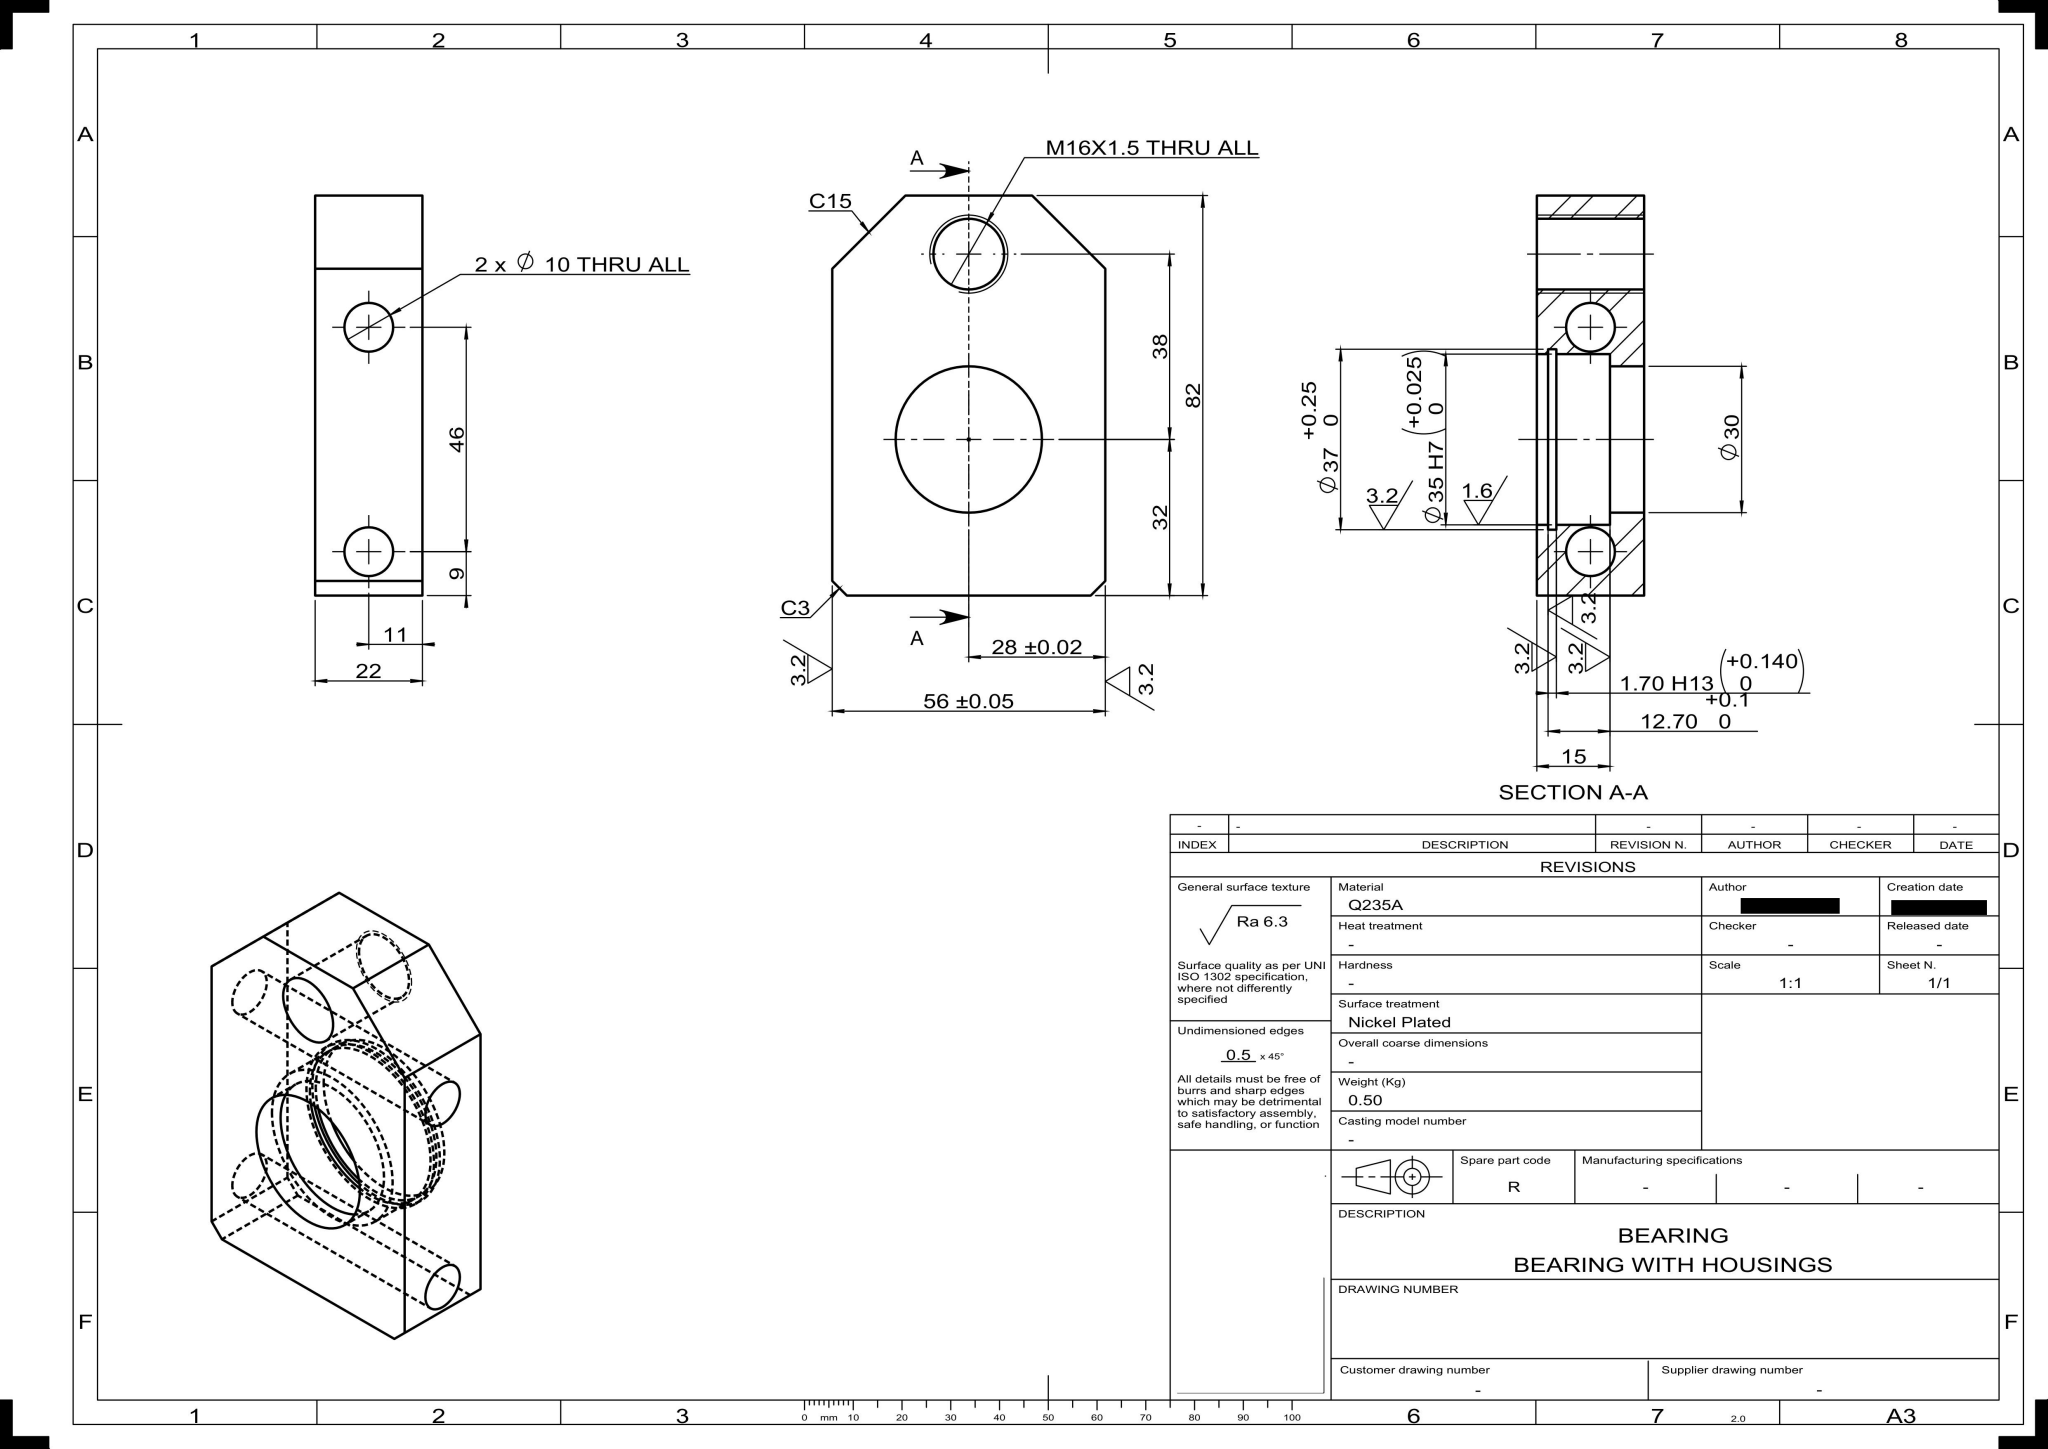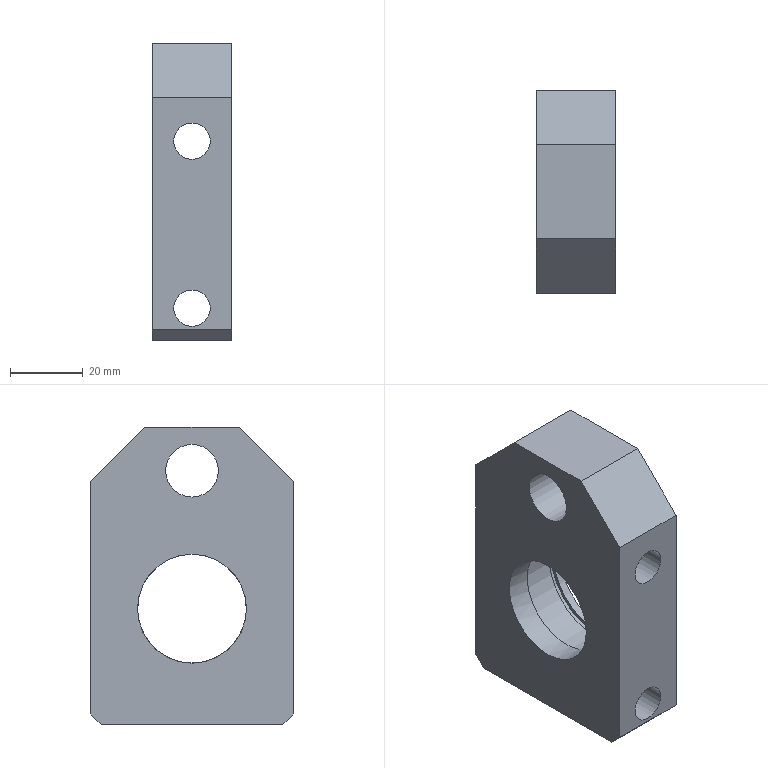Part | NX | mm | 1 solid | 20 faces | box 22 x 56 x 82 mm | volume 63875 mm3 | plane 13 | cylinder 7 | commonest cylinder face diameters 35 x2 10 x2 14.5 x1 30 x1 37 x1
STEP:
#1=CARTESIAN_POINT('',(0.,0.,0.));
#2=DIRECTION('',(0.,0.,1.));
#3=DIRECTION('',(1.,0.,0.));
#4=AXIS2_PLACEMENT_3D('',#1,#2,#3);
#5=(LENGTH_UNIT()NAMED_UNIT(*)SI_UNIT(.MILLI.,.METRE.));
#6=UNCERTAINTY_MEASURE_WITH_UNIT(LENGTH_MEASURE(0.00002),#5,'','');
#7=(NAMED_UNIT(*)PLANE_ANGLE_UNIT()SI_UNIT($,.RADIAN.));
#8=PLANE_ANGLE_MEASURE_WITH_UNIT(PLANE_ANGLE_MEASURE(0.01745),#7);
#9=DIMENSIONAL_EXPONENTS(0.,0.,0.,0.,0.,0.,0.);
#10=(CONVERSION_BASED_UNIT('',#8)NAMED_UNIT(#9)PLANE_ANGLE_UNIT());
#11=(NAMED_UNIT(*)SI_UNIT($,.STERADIAN.)SOLID_ANGLE_UNIT());
#12=(GEOMETRIC_REPRESENTATION_CONTEXT(3)GLOBAL_UNCERTAINTY_ASSIGNED_CONTEXT((#6))GLOBAL_UNIT_ASSIGNED_CONTEXT((#5,#10,#11))REPRESENTATION_CONTEXT('',''));
#13=SHAPE_REPRESENTATION('',(#4),#12);
#14=CARTESIAN_POINT('',(-4.,0.,14.5));
#15=VERTEX_POINT('',#14);
#16=CARTESIAN_POINT('',(-4.,0.,32.));
#17=DIRECTION('',(1.,0.,0.));
#18=DIRECTION('',(0.,0.,-1.));
#19=AXIS2_PLACEMENT_3D('',#16,#17,#18);
#20=CIRCLE('',#19,17.5);
#21=EDGE_CURVE('',#15,#15,#20,.T.);
#22=ORIENTED_EDGE('',*,*,#21,.F.);
#23=EDGE_LOOP('',(#22));
#24=FACE_BOUND('',#23,.T.);
#25=CARTESIAN_POINT('',(-4.,0.,13.5));
#26=VERTEX_POINT('',#25);
#27=CARTESIAN_POINT('',(-4.,0.,32.));
#28=DIRECTION('',(-1.,0.,0.));
#29=DIRECTION('',(0.,0.,-1.));
#30=AXIS2_PLACEMENT_3D('',#27,#28,#29);
#31=CIRCLE('',#30,18.5);
#32=EDGE_CURVE('',#26,#26,#31,.T.);
#33=ORIENTED_EDGE('',*,*,#32,.F.);
#34=EDGE_LOOP('',(#33));
#35=FACE_BOUND('',#34,.T.);
#36=CARTESIAN_POINT('',(-4.,0.,41.));
#37=DIRECTION('',(1.,0.,0.));
#38=DIRECTION('',(0.,0.,-1.));
#39=AXIS2_PLACEMENT_3D('',#36,#37,#38);
#40=PLANE('',#39);
#41=ADVANCED_FACE('',(#24,#35),#40,.T.);
#42=CARTESIAN_POINT('',(-11.,-28.,60.));
#43=VERTEX_POINT('',#42);
#44=CARTESIAN_POINT('',(-11.,-28.,55.));
#45=DIRECTION('',(0.,1.,0.));
#46=DIRECTION('',(0.,0.,1.));
#47=AXIS2_PLACEMENT_3D('',#44,#45,#46);
#48=CIRCLE('',#47,5.);
#49=EDGE_CURVE('',#43,#43,#48,.T.);
#50=ORIENTED_EDGE('',*,*,#49,.T.);
#51=EDGE_LOOP('',(#50));
#52=FACE_BOUND('',#51,.T.);
#53=CARTESIAN_POINT('',(-11.,-28.,14.));
#54=VERTEX_POINT('',#53);
#55=CARTESIAN_POINT('',(-11.,-28.,9.));
#56=DIRECTION('',(0.,1.,0.));
#57=DIRECTION('',(0.,0.,1.));
#58=AXIS2_PLACEMENT_3D('',#55,#56,#57);
#59=CIRCLE('',#58,5.);
#60=EDGE_CURVE('',#54,#54,#59,.T.);
#61=ORIENTED_EDGE('',*,*,#60,.T.);
#62=EDGE_LOOP('',(#61));
#63=FACE_BOUND('',#62,.T.);
#64=CARTESIAN_POINT('',(0.,-28.,67.));
#65=VERTEX_POINT('',#64);
#66=CARTESIAN_POINT('',(0.,-28.,3.));
#67=VERTEX_POINT('',#66);
#68=CARTESIAN_POINT('',(0.,-28.,82.));
#69=DIRECTION('',(0.,0.,-1.));
#70=VECTOR('',#69,1.);
#71=LINE('',#68,#70);
#72=EDGE_CURVE('',#65,#67,#71,.T.);
#73=ORIENTED_EDGE('',*,*,#72,.F.);
#74=CARTESIAN_POINT('',(-22.,-28.,67.));
#75=VERTEX_POINT('',#74);
#76=CARTESIAN_POINT('',(-22.,-28.,67.));
#77=DIRECTION('',(-1.,0.,0.));
#78=VECTOR('',#77,1.);
#79=LINE('',#76,#78);
#80=EDGE_CURVE('',#65,#75,#79,.T.);
#81=ORIENTED_EDGE('',*,*,#80,.T.);
#82=CARTESIAN_POINT('',(-22.,-28.,3.));
#83=VERTEX_POINT('',#82);
#84=CARTESIAN_POINT('',(-22.,-28.,82.));
#85=DIRECTION('',(0.,0.,-1.));
#86=VECTOR('',#85,1.);
#87=LINE('',#84,#86);
#88=EDGE_CURVE('',#75,#83,#87,.T.);
#89=ORIENTED_EDGE('',*,*,#88,.T.);
#90=CARTESIAN_POINT('',(-22.,-28.,3.));
#91=DIRECTION('',(1.,0.,0.));
#92=VECTOR('',#91,1.);
#93=LINE('',#90,#92);
#94=EDGE_CURVE('',#83,#67,#93,.T.);
#95=ORIENTED_EDGE('',*,*,#94,.T.);
#96=EDGE_LOOP('',(#73,#81,#89,#95));
#97=FACE_BOUND('',#96,.T.);
#98=CARTESIAN_POINT('',(-22.,-28.,82.));
#99=DIRECTION('',(0.,-1.,0.));
#100=DIRECTION('',(0.,0.,-1.));
#101=AXIS2_PLACEMENT_3D('',#98,#99,#100);
#102=PLANE('',#101);
#103=ADVANCED_FACE('',(#52,#63,#97),#102,.T.);
#104=CARTESIAN_POINT('',(-22.,-25.,0.));
#105=VERTEX_POINT('',#104);
#106=CARTESIAN_POINT('',(-22.,25.,0.));
#107=VERTEX_POINT('',#106);
#108=CARTESIAN_POINT('',(-22.,-28.,0.));
#109=DIRECTION('',(0.,1.,0.));
#110=VECTOR('',#109,1.);
#111=LINE('',#108,#110);
#112=EDGE_CURVE('',#105,#107,#111,.T.);
#113=ORIENTED_EDGE('',*,*,#112,.T.);
#114=CARTESIAN_POINT('',(0.,25.,0.));
#115=VERTEX_POINT('',#114);
#116=CARTESIAN_POINT('',(-22.,25.,0.));
#117=DIRECTION('',(1.,0.,0.));
#118=VECTOR('',#117,1.);
#119=LINE('',#116,#118);
#120=EDGE_CURVE('',#107,#115,#119,.T.);
#121=ORIENTED_EDGE('',*,*,#120,.T.);
#122=CARTESIAN_POINT('',(0.,-25.,0.));
#123=VERTEX_POINT('',#122);
#124=CARTESIAN_POINT('',(0.,-28.,0.));
#125=DIRECTION('',(0.,1.,0.));
#126=VECTOR('',#125,1.);
#127=LINE('',#124,#126);
#128=EDGE_CURVE('',#123,#115,#127,.T.);
#129=ORIENTED_EDGE('',*,*,#128,.F.);
#130=CARTESIAN_POINT('',(-22.,-25.,0.));
#131=DIRECTION('',(-1.,0.,0.));
#132=VECTOR('',#131,1.);
#133=LINE('',#130,#132);
#134=EDGE_CURVE('',#123,#105,#133,.T.);
#135=ORIENTED_EDGE('',*,*,#134,.T.);
#136=EDGE_LOOP('',(#113,#121,#129,#135));
#137=FACE_OUTER_BOUND('',#136,.T.);
#138=CARTESIAN_POINT('',(-22.,-28.,0.));
#139=DIRECTION('',(0.,0.,-1.));
#140=DIRECTION('',(-1.,0.,0.));
#141=AXIS2_PLACEMENT_3D('',#138,#139,#140);
#142=PLANE('',#141);
#143=ADVANCED_FACE('',(#137),#142,.T.);
#144=CARTESIAN_POINT('',(-11.,28.,60.));
#145=VERTEX_POINT('',#144);
#146=CARTESIAN_POINT('',(-11.,28.,55.));
#147=DIRECTION('',(0.,1.,0.));
#148=DIRECTION('',(0.,0.,1.));
#149=AXIS2_PLACEMENT_3D('',#146,#147,#148);
#150=CIRCLE('',#149,5.);
#151=EDGE_CURVE('',#145,#145,#150,.T.);
#152=ORIENTED_EDGE('',*,*,#151,.F.);
#153=EDGE_LOOP('',(#152));
#154=FACE_BOUND('',#153,.T.);
#155=CARTESIAN_POINT('',(-11.,28.,14.));
#156=VERTEX_POINT('',#155);
#157=CARTESIAN_POINT('',(-11.,28.,9.));
#158=DIRECTION('',(0.,1.,0.));
#159=DIRECTION('',(0.,0.,1.));
#160=AXIS2_PLACEMENT_3D('',#157,#158,#159);
#161=CIRCLE('',#160,5.);
#162=EDGE_CURVE('',#156,#156,#161,.T.);
#163=ORIENTED_EDGE('',*,*,#162,.F.);
#164=EDGE_LOOP('',(#163));
#165=FACE_BOUND('',#164,.T.);
#166=CARTESIAN_POINT('',(-22.,28.,3.));
#167=VERTEX_POINT('',#166);
#168=CARTESIAN_POINT('',(-22.,28.,67.));
#169=VERTEX_POINT('',#168);
#170=CARTESIAN_POINT('',(-22.,28.,0.));
#171=DIRECTION('',(0.,0.,1.));
#172=VECTOR('',#171,1.);
#173=LINE('',#170,#172);
#174=EDGE_CURVE('',#167,#169,#173,.T.);
#175=ORIENTED_EDGE('',*,*,#174,.T.);
#176=CARTESIAN_POINT('',(0.,28.,67.));
#177=VERTEX_POINT('',#176);
#178=CARTESIAN_POINT('',(-22.,28.,67.));
#179=DIRECTION('',(1.,0.,0.));
#180=VECTOR('',#179,1.);
#181=LINE('',#178,#180);
#182=EDGE_CURVE('',#169,#177,#181,.T.);
#183=ORIENTED_EDGE('',*,*,#182,.T.);
#184=CARTESIAN_POINT('',(0.,28.,3.));
#185=VERTEX_POINT('',#184);
#186=CARTESIAN_POINT('',(0.,28.,0.));
#187=DIRECTION('',(0.,0.,1.));
#188=VECTOR('',#187,1.);
#189=LINE('',#186,#188);
#190=EDGE_CURVE('',#185,#177,#189,.T.);
#191=ORIENTED_EDGE('',*,*,#190,.F.);
#192=CARTESIAN_POINT('',(-22.,28.,3.));
#193=DIRECTION('',(-1.,0.,0.));
#194=VECTOR('',#193,1.);
#195=LINE('',#192,#194);
#196=EDGE_CURVE('',#185,#167,#195,.T.);
#197=ORIENTED_EDGE('',*,*,#196,.T.);
#198=EDGE_LOOP('',(#175,#183,#191,#197));
#199=FACE_BOUND('',#198,.T.);
#200=CARTESIAN_POINT('',(-22.,28.,0.));
#201=DIRECTION('',(0.,1.,0.));
#202=DIRECTION('',(0.,0.,1.));
#203=AXIS2_PLACEMENT_3D('',#200,#201,#202);
#204=PLANE('',#203);
#205=ADVANCED_FACE('',(#154,#165,#199),#204,.T.);
#206=CARTESIAN_POINT('',(0.,13.,82.));
#207=VERTEX_POINT('',#206);
#208=CARTESIAN_POINT('',(0.,-13.,82.));
#209=VERTEX_POINT('',#208);
#210=CARTESIAN_POINT('',(0.,28.,82.));
#211=DIRECTION('',(0.,-1.,0.));
#212=VECTOR('',#211,1.);
#213=LINE('',#210,#212);
#214=EDGE_CURVE('',#207,#209,#213,.T.);
#215=ORIENTED_EDGE('',*,*,#214,.F.);
#216=CARTESIAN_POINT('',(-22.,13.,82.));
#217=VERTEX_POINT('',#216);
#218=CARTESIAN_POINT('',(-22.,13.,82.));
#219=DIRECTION('',(-1.,0.,0.));
#220=VECTOR('',#219,1.);
#221=LINE('',#218,#220);
#222=EDGE_CURVE('',#207,#217,#221,.T.);
#223=ORIENTED_EDGE('',*,*,#222,.T.);
#224=CARTESIAN_POINT('',(-22.,-13.,82.));
#225=VERTEX_POINT('',#224);
#226=CARTESIAN_POINT('',(-22.,28.,82.));
#227=DIRECTION('',(0.,-1.,0.));
#228=VECTOR('',#227,1.);
#229=LINE('',#226,#228);
#230=EDGE_CURVE('',#217,#225,#229,.T.);
#231=ORIENTED_EDGE('',*,*,#230,.T.);
#232=CARTESIAN_POINT('',(-22.,-13.,82.));
#233=DIRECTION('',(1.,0.,0.));
#234=VECTOR('',#233,1.);
#235=LINE('',#232,#234);
#236=EDGE_CURVE('',#225,#209,#235,.T.);
#237=ORIENTED_EDGE('',*,*,#236,.T.);
#238=EDGE_LOOP('',(#215,#223,#231,#237));
#239=FACE_OUTER_BOUND('',#238,.T.);
#240=CARTESIAN_POINT('',(-22.,28.,82.));
#241=DIRECTION('',(0.,0.,1.));
#242=DIRECTION('',(1.,0.,0.));
#243=AXIS2_PLACEMENT_3D('',#240,#241,#242);
#244=PLANE('',#243);
#245=ADVANCED_FACE('',(#239),#244,.T.);
#246=CARTESIAN_POINT('',(-22.,0.,62.75));
#247=VERTEX_POINT('',#246);
#248=CARTESIAN_POINT('',(-22.,0.,70.));
#249=DIRECTION('',(1.,0.,0.));
#250=DIRECTION('',(0.,0.,-1.));
#251=AXIS2_PLACEMENT_3D('',#248,#249,#250);
#252=CIRCLE('',#251,7.25);
#253=EDGE_CURVE('',#247,#247,#252,.T.);
#254=ORIENTED_EDGE('',*,*,#253,.F.);
#255=EDGE_LOOP('',(#254));
#256=FACE_BOUND('',#255,.T.);
#257=CARTESIAN_POINT('',(0.,0.,77.25));
#258=VERTEX_POINT('',#257);
#259=CARTESIAN_POINT('',(0.,0.,70.));
#260=DIRECTION('',(-1.,0.,0.));
#261=DIRECTION('',(0.,0.,1.));
#262=AXIS2_PLACEMENT_3D('',#259,#260,#261);
#263=CIRCLE('',#262,7.25);
#264=EDGE_CURVE('',#258,#258,#263,.T.);
#265=ORIENTED_EDGE('',*,*,#264,.F.);
#266=EDGE_LOOP('',(#265));
#267=FACE_BOUND('',#266,.T.);
#268=CARTESIAN_POINT('',(0.,0.,70.));
#269=DIRECTION('',(-1.,0.,0.));
#270=DIRECTION('',(0.,0.,1.));
#271=AXIS2_PLACEMENT_3D('',#268,#269,#270);
#272=CYLINDRICAL_SURFACE('',#271,7.25);
#273=ADVANCED_FACE('',(#256,#267),#272,.F.);
#274=CARTESIAN_POINT('',(-15.,0.,49.5));
#275=VERTEX_POINT('',#274);
#276=CARTESIAN_POINT('',(-15.,0.,32.));
#277=DIRECTION('',(1.,0.,0.));
#278=DIRECTION('',(0.,0.,1.));
#279=AXIS2_PLACEMENT_3D('',#276,#277,#278);
#280=CIRCLE('',#279,17.5);
#281=EDGE_CURVE('',#275,#275,#280,.T.);
#282=ORIENTED_EDGE('',*,*,#281,.F.);
#283=EDGE_LOOP('',(#282));
#284=FACE_BOUND('',#283,.T.);
#285=ORIENTED_EDGE('',*,*,#21,.T.);
#286=EDGE_LOOP('',(#285));
#287=FACE_BOUND('',#286,.T.);
#288=CARTESIAN_POINT('',(-0.,0.,32.));
#289=DIRECTION('',(-1.,0.,0.));
#290=DIRECTION('',(0.,0.,1.));
#291=AXIS2_PLACEMENT_3D('',#288,#289,#290);
#292=CYLINDRICAL_SURFACE('',#291,17.5);
#293=ADVANCED_FACE('',(#284,#287),#292,.F.);
#294=CARTESIAN_POINT('',(-22.,0.,17.));
#295=VERTEX_POINT('',#294);
#296=CARTESIAN_POINT('',(-22.,0.,32.));
#297=DIRECTION('',(1.,0.,0.));
#298=DIRECTION('',(0.,0.,-1.));
#299=AXIS2_PLACEMENT_3D('',#296,#297,#298);
#300=CIRCLE('',#299,15.);
#301=EDGE_CURVE('',#295,#295,#300,.T.);
#302=ORIENTED_EDGE('',*,*,#301,.T.);
#303=EDGE_LOOP('',(#302));
#304=FACE_BOUND('',#303,.T.);
#305=ORIENTED_EDGE('',*,*,#253,.T.);
#306=EDGE_LOOP('',(#305));
#307=FACE_BOUND('',#306,.T.);
#308=ORIENTED_EDGE('',*,*,#230,.F.);
#309=CARTESIAN_POINT('',(-22.,28.,67.));
#310=DIRECTION('',(0.,0.7071,-0.7071));
#311=VECTOR('',#310,1.);
#312=LINE('',#309,#311);
#313=EDGE_CURVE('',#217,#169,#312,.T.);
#314=ORIENTED_EDGE('',*,*,#313,.T.);
#315=ORIENTED_EDGE('',*,*,#174,.F.);
#316=CARTESIAN_POINT('',(-22.,25.,0.));
#317=DIRECTION('',(0.,-0.7071,-0.7071));
#318=VECTOR('',#317,1.);
#319=LINE('',#316,#318);
#320=EDGE_CURVE('',#167,#107,#319,.T.);
#321=ORIENTED_EDGE('',*,*,#320,.T.);
#322=ORIENTED_EDGE('',*,*,#112,.F.);
#323=CARTESIAN_POINT('',(-22.,-28.,3.));
#324=DIRECTION('',(0.,-0.7071,0.7071));
#325=VECTOR('',#324,1.);
#326=LINE('',#323,#325);
#327=EDGE_CURVE('',#105,#83,#326,.T.);
#328=ORIENTED_EDGE('',*,*,#327,.T.);
#329=ORIENTED_EDGE('',*,*,#88,.F.);
#330=CARTESIAN_POINT('',(-22.,-13.,82.));
#331=DIRECTION('',(0.,0.7071,0.7071));
#332=VECTOR('',#331,1.);
#333=LINE('',#330,#332);
#334=EDGE_CURVE('',#75,#225,#333,.T.);
#335=ORIENTED_EDGE('',*,*,#334,.T.);
#336=EDGE_LOOP('',(#308,#314,#315,#321,#322,#328,#329,#335));
#337=FACE_BOUND('',#336,.T.);
#338=CARTESIAN_POINT('',(-22.,0.,0.));
#339=DIRECTION('',(1.,0.,0.));
#340=DIRECTION('',(0.,0.,-1.));
#341=AXIS2_PLACEMENT_3D('',#338,#339,#340);
#342=PLANE('',#341);
#343=ADVANCED_FACE('',(#304,#307,#337),#342,.F.);
#344=CARTESIAN_POINT('',(-15.,0.,47.));
#345=VERTEX_POINT('',#344);
#346=CARTESIAN_POINT('',(-15.,0.,32.));
#347=DIRECTION('',(1.,0.,0.));
#348=DIRECTION('',(0.,0.,1.));
#349=AXIS2_PLACEMENT_3D('',#346,#347,#348);
#350=CIRCLE('',#349,15.);
#351=EDGE_CURVE('',#345,#345,#350,.T.);
#352=ORIENTED_EDGE('',*,*,#351,.T.);
#353=EDGE_LOOP('',(#352));
#354=FACE_BOUND('',#353,.T.);
#355=ORIENTED_EDGE('',*,*,#301,.F.);
#356=EDGE_LOOP('',(#355));
#357=FACE_BOUND('',#356,.T.);
#358=CARTESIAN_POINT('',(-66.209,0.,32.));
#359=DIRECTION('',(-1.,0.,0.));
#360=DIRECTION('',(0.,0.,1.));
#361=AXIS2_PLACEMENT_3D('',#358,#359,#360);
#362=CYLINDRICAL_SURFACE('',#361,15.);
#363=ADVANCED_FACE('',(#354,#357),#362,.F.);
#364=ORIENTED_EDGE('',*,*,#351,.F.);
#365=EDGE_LOOP('',(#364));
#366=FACE_BOUND('',#365,.T.);
#367=ORIENTED_EDGE('',*,*,#281,.T.);
#368=EDGE_LOOP('',(#367));
#369=FACE_BOUND('',#368,.T.);
#370=CARTESIAN_POINT('',(-15.,0.,32.));
#371=DIRECTION('',(-1.,0.,0.));
#372=DIRECTION('',(0.,0.,1.));
#373=AXIS2_PLACEMENT_3D('',#370,#371,#372);
#374=PLANE('',#373);
#375=ADVANCED_FACE('',(#366,#369),#374,.F.);
#376=CARTESIAN_POINT('',(-2.3,0.,14.5));
#377=VERTEX_POINT('',#376);
#378=CARTESIAN_POINT('',(-2.3,0.,32.));
#379=DIRECTION('',(-1.,0.,0.));
#380=DIRECTION('',(0.,0.,-1.));
#381=AXIS2_PLACEMENT_3D('',#378,#379,#380);
#382=CIRCLE('',#381,17.5);
#383=EDGE_CURVE('',#377,#377,#382,.T.);
#384=ORIENTED_EDGE('',*,*,#383,.F.);
#385=EDGE_LOOP('',(#384));
#386=FACE_BOUND('',#385,.T.);
#387=CARTESIAN_POINT('',(-2.3,0.,13.5));
#388=VERTEX_POINT('',#387);
#389=CARTESIAN_POINT('',(-2.3,0.,32.));
#390=DIRECTION('',(1.,0.,0.));
#391=DIRECTION('',(0.,0.,-1.));
#392=AXIS2_PLACEMENT_3D('',#389,#390,#391);
#393=CIRCLE('',#392,18.5);
#394=EDGE_CURVE('',#388,#388,#393,.T.);
#395=ORIENTED_EDGE('',*,*,#394,.F.);
#396=EDGE_LOOP('',(#395));
#397=FACE_BOUND('',#396,.T.);
#398=CARTESIAN_POINT('',(-2.3,0.,32.));
#399=DIRECTION('',(1.,0.,0.));
#400=DIRECTION('',(0.,0.,-1.));
#401=AXIS2_PLACEMENT_3D('',#398,#399,#400);
#402=PLANE('',#401);
#403=ADVANCED_FACE('',(#386,#397),#402,.F.);
#404=CARTESIAN_POINT('',(-0.,0.,49.5));
#405=VERTEX_POINT('',#404);
#406=CARTESIAN_POINT('',(-0.,0.,32.));
#407=DIRECTION('',(-1.,0.,0.));
#408=DIRECTION('',(0.,0.,1.));
#409=AXIS2_PLACEMENT_3D('',#406,#407,#408);
#410=CIRCLE('',#409,17.5);
#411=EDGE_CURVE('',#405,#405,#410,.T.);
#412=ORIENTED_EDGE('',*,*,#411,.T.);
#413=EDGE_LOOP('',(#412));
#414=FACE_BOUND('',#413,.T.);
#415=ORIENTED_EDGE('',*,*,#264,.T.);
#416=EDGE_LOOP('',(#415));
#417=FACE_BOUND('',#416,.T.);
#418=ORIENTED_EDGE('',*,*,#190,.T.);
#419=CARTESIAN_POINT('',(0.,47.5,47.5));
#420=DIRECTION('',(0.,-0.7071,0.7071));
#421=VECTOR('',#420,1.);
#422=LINE('',#419,#421);
#423=EDGE_CURVE('',#177,#207,#422,.T.);
#424=ORIENTED_EDGE('',*,*,#423,.T.);
#425=ORIENTED_EDGE('',*,*,#214,.T.);
#426=CARTESIAN_POINT('',(0.,-47.5,47.5));
#427=DIRECTION('',(0.,-0.7071,-0.7071));
#428=VECTOR('',#427,1.);
#429=LINE('',#426,#428);
#430=EDGE_CURVE('',#209,#65,#429,.T.);
#431=ORIENTED_EDGE('',*,*,#430,.T.);
#432=ORIENTED_EDGE('',*,*,#72,.T.);
#433=CARTESIAN_POINT('',(0.,-12.5,-12.5));
#434=DIRECTION('',(0.,0.7071,-0.7071));
#435=VECTOR('',#434,1.);
#436=LINE('',#433,#435);
#437=EDGE_CURVE('',#67,#123,#436,.T.);
#438=ORIENTED_EDGE('',*,*,#437,.T.);
#439=ORIENTED_EDGE('',*,*,#128,.T.);
#440=CARTESIAN_POINT('',(0.,12.5,-12.5));
#441=DIRECTION('',(0.,0.7071,0.7071));
#442=VECTOR('',#441,1.);
#443=LINE('',#440,#442);
#444=EDGE_CURVE('',#115,#185,#443,.T.);
#445=ORIENTED_EDGE('',*,*,#444,.T.);
#446=EDGE_LOOP('',(#418,#424,#425,#431,#432,#438,#439,#445));
#447=FACE_BOUND('',#446,.T.);
#448=CARTESIAN_POINT('',(0.,0.,0.));
#449=DIRECTION('',(1.,0.,0.));
#450=DIRECTION('',(0.,0.,-1.));
#451=AXIS2_PLACEMENT_3D('',#448,#449,#450);
#452=PLANE('',#451);
#453=ADVANCED_FACE('',(#414,#417,#447),#452,.T.);
#454=ORIENTED_EDGE('',*,*,#383,.T.);
#455=EDGE_LOOP('',(#454));
#456=FACE_BOUND('',#455,.T.);
#457=ORIENTED_EDGE('',*,*,#411,.F.);
#458=EDGE_LOOP('',(#457));
#459=FACE_BOUND('',#458,.T.);
#460=CARTESIAN_POINT('',(-0.,0.,32.));
#461=DIRECTION('',(-1.,0.,0.));
#462=DIRECTION('',(0.,0.,1.));
#463=AXIS2_PLACEMENT_3D('',#460,#461,#462);
#464=CYLINDRICAL_SURFACE('',#463,17.5);
#465=ADVANCED_FACE('',(#456,#459),#464,.F.);
#466=ORIENTED_EDGE('',*,*,#32,.T.);
#467=EDGE_LOOP('',(#466));
#468=FACE_BOUND('',#467,.T.);
#469=ORIENTED_EDGE('',*,*,#394,.T.);
#470=EDGE_LOOP('',(#469));
#471=FACE_BOUND('',#470,.T.);
#472=CARTESIAN_POINT('',(-0.,0.,32.));
#473=DIRECTION('',(-1.,0.,0.));
#474=DIRECTION('',(0.,0.,1.));
#475=AXIS2_PLACEMENT_3D('',#472,#473,#474);
#476=CYLINDRICAL_SURFACE('',#475,18.5);
#477=ADVANCED_FACE('',(#468,#471),#476,.F.);
#478=ORIENTED_EDGE('',*,*,#162,.T.);
#479=EDGE_LOOP('',(#478));
#480=FACE_BOUND('',#479,.T.);
#481=ORIENTED_EDGE('',*,*,#60,.F.);
#482=EDGE_LOOP('',(#481));
#483=FACE_BOUND('',#482,.T.);
#484=CARTESIAN_POINT('',(-11.,-28.,9.));
#485=DIRECTION('',(0.,1.,0.));
#486=DIRECTION('',(0.,0.,1.));
#487=AXIS2_PLACEMENT_3D('',#484,#485,#486);
#488=CYLINDRICAL_SURFACE('',#487,5.);
#489=ADVANCED_FACE('',(#480,#483),#488,.F.);
#490=ORIENTED_EDGE('',*,*,#151,.T.);
#491=EDGE_LOOP('',(#490));
#492=FACE_BOUND('',#491,.T.);
#493=ORIENTED_EDGE('',*,*,#49,.F.);
#494=EDGE_LOOP('',(#493));
#495=FACE_BOUND('',#494,.T.);
#496=CARTESIAN_POINT('',(-11.,-28.,55.));
#497=DIRECTION('',(0.,1.,0.));
#498=DIRECTION('',(0.,0.,1.));
#499=AXIS2_PLACEMENT_3D('',#496,#497,#498);
#500=CYLINDRICAL_SURFACE('',#499,5.);
#501=ADVANCED_FACE('',(#492,#495),#500,.F.);
#502=ORIENTED_EDGE('',*,*,#313,.F.);
#503=ORIENTED_EDGE('',*,*,#222,.F.);
#504=ORIENTED_EDGE('',*,*,#423,.F.);
#505=ORIENTED_EDGE('',*,*,#182,.F.);
#506=EDGE_LOOP('',(#502,#503,#504,#505));
#507=FACE_OUTER_BOUND('',#506,.T.);
#508=CARTESIAN_POINT('',(-22.,28.,67.));
#509=DIRECTION('',(0.,-0.7071,-0.7071));
#510=DIRECTION('',(1.,0.,0.));
#511=AXIS2_PLACEMENT_3D('',#508,#509,#510);
#512=PLANE('',#511);
#513=ADVANCED_FACE('',(#507),#512,.F.);
#514=ORIENTED_EDGE('',*,*,#334,.F.);
#515=ORIENTED_EDGE('',*,*,#80,.F.);
#516=ORIENTED_EDGE('',*,*,#430,.F.);
#517=ORIENTED_EDGE('',*,*,#236,.F.);
#518=EDGE_LOOP('',(#514,#515,#516,#517));
#519=FACE_OUTER_BOUND('',#518,.T.);
#520=CARTESIAN_POINT('',(-22.,-13.,82.));
#521=DIRECTION('',(0.,0.7071,-0.7071));
#522=DIRECTION('',(1.,0.,0.));
#523=AXIS2_PLACEMENT_3D('',#520,#521,#522);
#524=PLANE('',#523);
#525=ADVANCED_FACE('',(#519),#524,.F.);
#526=ORIENTED_EDGE('',*,*,#320,.F.);
#527=ORIENTED_EDGE('',*,*,#196,.F.);
#528=ORIENTED_EDGE('',*,*,#444,.F.);
#529=ORIENTED_EDGE('',*,*,#120,.F.);
#530=EDGE_LOOP('',(#526,#527,#528,#529));
#531=FACE_OUTER_BOUND('',#530,.T.);
#532=CARTESIAN_POINT('',(-22.,25.,0.));
#533=DIRECTION('',(0.,-0.7071,0.7071));
#534=DIRECTION('',(1.,0.,0.));
#535=AXIS2_PLACEMENT_3D('',#532,#533,#534);
#536=PLANE('',#535);
#537=ADVANCED_FACE('',(#531),#536,.F.);
#538=ORIENTED_EDGE('',*,*,#327,.F.);
#539=ORIENTED_EDGE('',*,*,#134,.F.);
#540=ORIENTED_EDGE('',*,*,#437,.F.);
#541=ORIENTED_EDGE('',*,*,#94,.F.);
#542=EDGE_LOOP('',(#538,#539,#540,#541));
#543=FACE_OUTER_BOUND('',#542,.T.);
#544=CARTESIAN_POINT('',(-22.,-28.,3.));
#545=DIRECTION('',(0.,0.7071,0.7071));
#546=DIRECTION('',(1.,0.,0.));
#547=AXIS2_PLACEMENT_3D('',#544,#545,#546);
#548=PLANE('',#547);
#549=ADVANCED_FACE('',(#543),#548,.F.);
#550=CLOSED_SHELL('',(#41,#103,#143,#205,#245,#273,#293,#343,#363,#375,#403,#453,#465,#477,#489,#501,#513,#525,#537,#549));
#551=MANIFOLD_SOLID_BREP('',#550);
#552=ADVANCED_BREP_SHAPE_REPRESENTATION('',(#551),#12);
#553=SHAPE_REPRESENTATION_RELATIONSHIP('','',#13,#552);
#554=PRESENTATION_LAYER_ASSIGNMENT('','',(#551));
#555=COLOUR_RGB('',0.4,0.8,1.);
#556=FILL_AREA_STYLE_COLOUR('',#555);
#557=FILL_AREA_STYLE('',(#556));
#558=SURFACE_STYLE_FILL_AREA(#557);
#559=SURFACE_SIDE_STYLE('',(#558));
#560=SURFACE_STYLE_USAGE(.BOTH.,#559);
#561=PRESENTATION_STYLE_ASSIGNMENT((#560));
#562=STYLED_ITEM('',(#561),#551);
#563=MECHANICAL_DESIGN_GEOMETRIC_PRESENTATION_REPRESENTATION('',(#562),#12);